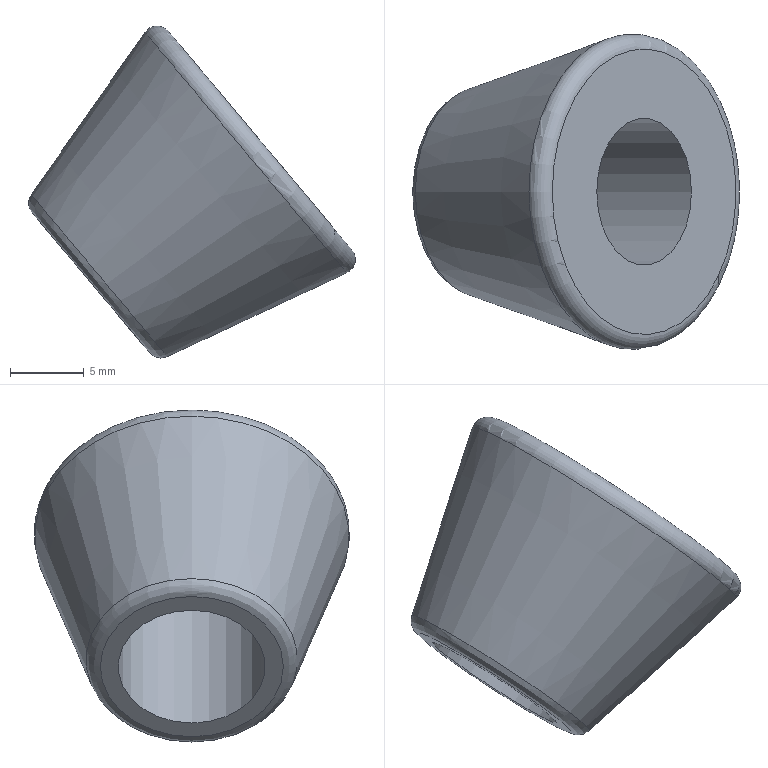Component | NX | HANGERBUSHING | 1 solid | 6 faces | box 22.19 x 21.39 x 22.54 mm | volume 2664 mm3 | plane 2 | torus 2 | cone 1 | cylinder 1 | commonest cylinder face diameters 10 x1
STEP:
#1=CARTESIAN_POINT('',(0.,0.,0.));
#2=DIRECTION('',(0.,0.,1.));
#3=DIRECTION('',(1.,0.,0.));
#4=AXIS2_PLACEMENT_3D('',#1,#2,#3);
#5=CARTESIAN_POINT('',(-451.275,-0.,-55.009));
#6=VERTEX_POINT('',#5);
#7=CARTESIAN_POINT('',(-446.66,-0.,-60.509));
#8=DIRECTION('',(0.766,0.,0.6428));
#9=DIRECTION('',(-0.6428,0.,0.766));
#10=AXIS2_PLACEMENT_3D('',#7,#8,#9);
#11=CIRCLE('',#10,7.179);
#12=CARTESIAN_POINT('',(-435.737,-0.,-51.344));
#13=DIRECTION('',(0.766,0.,0.6428));
#14=DIRECTION('',(-0.6428,0.,0.766));
#15=AXIS2_PLACEMENT_3D('',#12,#13,#14);
#16=CONICAL_SURFACE('',#15,11.,0.2618);
#17=CARTESIAN_POINT('',(0.,-14.259));
#18=DIRECTION('',(1.,0.));
#19=VECTOR('',#18,1.);
#20=LINE('',#17,#19);
#21=(GEOMETRIC_REPRESENTATION_CONTEXT(2)PARAMETRIC_REPRESENTATION_CONTEXT()REPRESENTATION_CONTEXT('',''));
#22=DEFINITIONAL_REPRESENTATION('',(#20),#21);
#23=PCURVE('',#16,#22);
#24=CARTESIAN_POINT('',(-446.462,-0.,-60.343));
#25=DIRECTION('',(0.766,0.,0.6428));
#26=DIRECTION('',(-0.6428,0.,0.766));
#27=AXIS2_PLACEMENT_3D('',#24,#25,#26);
#28=TOROIDAL_SURFACE('',#27,6.213,1.);
#29=CARTESIAN_POINT('',(0.,6.021));
#30=DIRECTION('',(1.,0.));
#31=VECTOR('',#30,1.);
#32=LINE('',#29,#31);
#33=(GEOMETRIC_REPRESENTATION_CONTEXT(2)PARAMETRIC_REPRESENTATION_CONTEXT()REPRESENTATION_CONTEXT('',''));
#34=DEFINITIONAL_REPRESENTATION('',(#32),#33);
#35=PCURVE('',#28,#34);
#36=SURFACE_CURVE('',#11,(#23,#35),.PCURVE_S1.);
#37=EDGE_CURVE('',#6,#6,#36,.T.);
#38=ORIENTED_EDGE('',*,*,#37,.T.);
#39=CARTESIAN_POINT('',(-443.555,-0.,-43.985));
#40=VERTEX_POINT('',#39);
#41=CARTESIAN_POINT('',(-451.275,-0.,-55.009));
#42=CARTESIAN_POINT('',(-443.555,-0.,-43.985));
#43=B_SPLINE_CURVE_WITH_KNOTS('',1,(#41,#42),.UNSPECIFIED.,.F.,.F.,(2,2),(-14.762,-1.303),.PIECEWISE_BEZIER_KNOTS.);
#44=CARTESIAN_POINT('',(6.283,0.));
#45=DIRECTION('',(0.,1.));
#46=VECTOR('',#45,1.);
#47=LINE('',#44,#46);
#48=(GEOMETRIC_REPRESENTATION_CONTEXT(2)PARAMETRIC_REPRESENTATION_CONTEXT()REPRESENTATION_CONTEXT('',''));
#49=DEFINITIONAL_REPRESENTATION('',(#47),#48);
#50=PCURVE('',#16,#49);
#51=CARTESIAN_POINT('',(0.,0.));
#52=DIRECTION('',(0.,1.));
#53=VECTOR('',#52,1.);
#54=LINE('',#51,#53);
#55=(GEOMETRIC_REPRESENTATION_CONTEXT(2)PARAMETRIC_REPRESENTATION_CONTEXT()REPRESENTATION_CONTEXT('',''));
#56=DEFINITIONAL_REPRESENTATION('',(#54),#55);
#57=PCURVE('',#16,#56);
#58=SEAM_CURVE('',#43,(#50,#57),.PCURVE_S1.);
#59=EDGE_CURVE('',#6,#40,#58,.T.);
#60=ORIENTED_EDGE('',*,*,#59,.T.);
#61=CARTESIAN_POINT('',(-429.848,-0.,-60.321));
#62=VERTEX_POINT('',#61);
#63=CARTESIAN_POINT('',(-436.702,-0.,-52.153));
#64=DIRECTION('',(-0.766,0.,-0.6428));
#65=DIRECTION('',(0.6428,0.,-0.766));
#66=AXIS2_PLACEMENT_3D('',#63,#64,#65);
#67=CIRCLE('',#66,10.663);
#68=CARTESIAN_POINT('',(9.425,-1.259));
#69=DIRECTION('',(-1.,0.));
#70=VECTOR('',#69,1.);
#71=LINE('',#68,#70);
#72=(GEOMETRIC_REPRESENTATION_CONTEXT(2)PARAMETRIC_REPRESENTATION_CONTEXT()REPRESENTATION_CONTEXT('',''));
#73=DEFINITIONAL_REPRESENTATION('',(#71),#72);
#74=PCURVE('',#16,#73);
#75=CARTESIAN_POINT('',(-436.503,-0.,-51.987));
#76=DIRECTION('',(0.766,0.,0.6428));
#77=DIRECTION('',(-0.6428,0.,0.766));
#78=AXIS2_PLACEMENT_3D('',#75,#76,#77);
#79=TOROIDAL_SURFACE('',#78,9.697,1.);
#80=CARTESIAN_POINT('',(9.425,6.021));
#81=DIRECTION('',(-1.,-0.));
#82=VECTOR('',#81,1.);
#83=LINE('',#80,#82);
#84=(GEOMETRIC_REPRESENTATION_CONTEXT(2)PARAMETRIC_REPRESENTATION_CONTEXT()REPRESENTATION_CONTEXT('',''));
#85=DEFINITIONAL_REPRESENTATION('',(#83),#84);
#86=PCURVE('',#79,#85);
#87=SURFACE_CURVE('',#67,(#74,#86),.PCURVE_S1.);
#88=EDGE_CURVE('',#40,#62,#87,.T.);
#89=ORIENTED_EDGE('',*,*,#88,.T.);
#90=CARTESIAN_POINT('',(-436.702,-0.,-52.153));
#91=DIRECTION('',(-0.766,0.,-0.6428));
#92=DIRECTION('',(0.6428,0.,-0.766));
#93=AXIS2_PLACEMENT_3D('',#90,#91,#92);
#94=CIRCLE('',#93,10.663);
#95=CARTESIAN_POINT('',(3.142,-1.259));
#96=DIRECTION('',(-1.,0.));
#97=VECTOR('',#96,1.);
#98=LINE('',#95,#97);
#99=(GEOMETRIC_REPRESENTATION_CONTEXT(2)PARAMETRIC_REPRESENTATION_CONTEXT()REPRESENTATION_CONTEXT('',''));
#100=DEFINITIONAL_REPRESENTATION('',(#98),#99);
#101=PCURVE('',#16,#100);
#102=CARTESIAN_POINT('',(3.142,6.021));
#103=DIRECTION('',(-1.,0.));
#104=VECTOR('',#103,1.);
#105=LINE('',#102,#104);
#106=(GEOMETRIC_REPRESENTATION_CONTEXT(2)PARAMETRIC_REPRESENTATION_CONTEXT()REPRESENTATION_CONTEXT('',''));
#107=DEFINITIONAL_REPRESENTATION('',(#105),#106);
#108=PCURVE('',#79,#107);
#109=SURFACE_CURVE('',#94,(#101,#108),.PCURVE_S1.);
#110=EDGE_CURVE('',#62,#40,#109,.T.);
#111=ORIENTED_EDGE('',*,*,#110,.T.);
#112=ORIENTED_EDGE('',*,*,#59,.F.);
#113=EDGE_LOOP('',(#38,#60,#89,#111,#112));
#114=FACE_BOUND('',#113,.T.);
#115=ADVANCED_FACE('',(#114),#16,.T.);
#116=CARTESIAN_POINT('',(-450.442,-0.,-57.155));
#117=VERTEX_POINT('',#116);
#118=CARTESIAN_POINT('',(-447.228,-0.,-60.986));
#119=DIRECTION('',(0.766,0.,0.6428));
#120=DIRECTION('',(-0.6428,0.,0.766));
#121=AXIS2_PLACEMENT_3D('',#118,#119,#120);
#122=CIRCLE('',#121,5.);
#123=CARTESIAN_POINT('',(-447.228,-0.,-60.986));
#124=DIRECTION('',(0.766,0.,0.6428));
#125=DIRECTION('',(-0.6428,0.,0.766));
#126=AXIS2_PLACEMENT_3D('',#123,#124,#125);
#127=PLANE('',#126);
#128=CARTESIAN_POINT('',(0.,0.));
#129=DIRECTION('',(1.,0.));
#130=AXIS2_PLACEMENT_2D('',#128,#129);
#131=CIRCLE('',#130,5.);
#132=(GEOMETRIC_REPRESENTATION_CONTEXT(2)PARAMETRIC_REPRESENTATION_CONTEXT()REPRESENTATION_CONTEXT('',''));
#133=DEFINITIONAL_REPRESENTATION('',(#131),#132);
#134=PCURVE('',#127,#133);
#135=CARTESIAN_POINT('',(-447.228,-0.,-60.986));
#136=DIRECTION('',(0.766,0.,0.6428));
#137=DIRECTION('',(-0.6428,0.,0.766));
#138=AXIS2_PLACEMENT_3D('',#135,#136,#137);
#139=CYLINDRICAL_SURFACE('',#138,5.);
#140=CARTESIAN_POINT('',(0.,0.));
#141=DIRECTION('',(1.,0.));
#142=VECTOR('',#141,1.);
#143=LINE('',#140,#142);
#144=(GEOMETRIC_REPRESENTATION_CONTEXT(2)PARAMETRIC_REPRESENTATION_CONTEXT()REPRESENTATION_CONTEXT('',''));
#145=DEFINITIONAL_REPRESENTATION('',(#143),#144);
#146=PCURVE('',#139,#145);
#147=SURFACE_CURVE('',#122,(#134,#146),.PCURVE_S1.);
#148=EDGE_CURVE('',#117,#117,#147,.T.);
#149=ORIENTED_EDGE('',*,*,#148,.T.);
#150=EDGE_LOOP('',(#149));
#151=FACE_BOUND('',#150,.T.);
#152=CARTESIAN_POINT('',(-451.222,-0.,-56.226));
#153=VERTEX_POINT('',#152);
#154=CARTESIAN_POINT('',(-447.228,-0.,-60.986));
#155=DIRECTION('',(-0.766,0.,-0.6428));
#156=DIRECTION('',(-0.6428,0.,0.766));
#157=AXIS2_PLACEMENT_3D('',#154,#155,#156);
#158=CIRCLE('',#157,6.213);
#159=CARTESIAN_POINT('',(6.213,0.));
#160=CARTESIAN_POINT('',(6.213,-10.762));
#161=CARTESIAN_POINT('',(-3.107,-5.381));
#162=CARTESIAN_POINT('',(-12.427,-0.));
#163=CARTESIAN_POINT('',(-3.107,5.381));
#164=CARTESIAN_POINT('',(6.213,10.762));
#165=CARTESIAN_POINT('',(6.213,0.));
#166=(BOUNDED_CURVE()B_SPLINE_CURVE(2,(#159,#160,#161,#162,#163,#164,#165),.UNSPECIFIED.,.T.,.F.)B_SPLINE_CURVE_WITH_KNOTS((1,2,2,2,2,1),(-2.094,0.,2.094,4.189,6.283,8.378),.UNSPECIFIED.)CURVE()GEOMETRIC_REPRESENTATION_ITEM()RATIONAL_B_SPLINE_CURVE((1.,0.5,1.,0.5,1.,0.5,1.))REPRESENTATION_ITEM(''));
#167=(GEOMETRIC_REPRESENTATION_CONTEXT(2)PARAMETRIC_REPRESENTATION_CONTEXT()REPRESENTATION_CONTEXT('',''));
#168=DEFINITIONAL_REPRESENTATION('',(#166),#167);
#169=PCURVE('',#127,#168);
#170=CARTESIAN_POINT('',(6.283,4.712));
#171=DIRECTION('',(-1.,0.));
#172=VECTOR('',#171,1.);
#173=LINE('',#170,#172);
#174=(GEOMETRIC_REPRESENTATION_CONTEXT(2)PARAMETRIC_REPRESENTATION_CONTEXT()REPRESENTATION_CONTEXT('',''));
#175=DEFINITIONAL_REPRESENTATION('',(#173),#174);
#176=PCURVE('',#28,#175);
#177=SURFACE_CURVE('',#158,(#169,#176),.PCURVE_S1.);
#178=EDGE_CURVE('',#153,#153,#177,.T.);
#179=ORIENTED_EDGE('',*,*,#178,.T.);
#180=EDGE_LOOP('',(#179));
#181=FACE_BOUND('',#180,.T.);
#182=ADVANCED_FACE('',(#151,#181),#127,.F.);
#183=CARTESIAN_POINT('',(-438.951,-0.,-47.514));
#184=VERTEX_POINT('',#183);
#185=CARTESIAN_POINT('',(-435.737,-0.,-51.344));
#186=DIRECTION('',(0.766,0.,0.6428));
#187=DIRECTION('',(-0.6428,0.,0.766));
#188=AXIS2_PLACEMENT_3D('',#185,#186,#187);
#189=CIRCLE('',#188,5.);
#190=CARTESIAN_POINT('',(-435.737,-0.,-51.344));
#191=DIRECTION('',(0.766,0.,0.6428));
#192=DIRECTION('',(-0.6428,0.,0.766));
#193=AXIS2_PLACEMENT_3D('',#190,#191,#192);
#194=PLANE('',#193);
#195=CARTESIAN_POINT('',(0.,0.));
#196=DIRECTION('',(1.,0.));
#197=AXIS2_PLACEMENT_2D('',#195,#196);
#198=CIRCLE('',#197,5.);
#199=(GEOMETRIC_REPRESENTATION_CONTEXT(2)PARAMETRIC_REPRESENTATION_CONTEXT()REPRESENTATION_CONTEXT('',''));
#200=DEFINITIONAL_REPRESENTATION('',(#198),#199);
#201=PCURVE('',#194,#200);
#202=CARTESIAN_POINT('',(0.,15.));
#203=DIRECTION('',(1.,0.));
#204=VECTOR('',#203,1.);
#205=LINE('',#202,#204);
#206=(GEOMETRIC_REPRESENTATION_CONTEXT(2)PARAMETRIC_REPRESENTATION_CONTEXT()REPRESENTATION_CONTEXT('',''));
#207=DEFINITIONAL_REPRESENTATION('',(#205),#206);
#208=PCURVE('',#139,#207);
#209=SURFACE_CURVE('',#189,(#201,#208),.PCURVE_S1.);
#210=EDGE_CURVE('',#184,#184,#209,.T.);
#211=ORIENTED_EDGE('',*,*,#210,.F.);
#212=EDGE_LOOP('',(#211));
#213=FACE_BOUND('',#212,.T.);
#214=CARTESIAN_POINT('',(-441.97,-0.,-43.916));
#215=VERTEX_POINT('',#214);
#216=CARTESIAN_POINT('',(-435.737,-0.,-51.344));
#217=DIRECTION('',(0.766,0.,0.6428));
#218=DIRECTION('',(-0.6428,0.,0.766));
#219=AXIS2_PLACEMENT_3D('',#216,#217,#218);
#220=CIRCLE('',#219,9.697);
#221=CARTESIAN_POINT('',(0.,0.));
#222=DIRECTION('',(1.,0.));
#223=AXIS2_PLACEMENT_2D('',#221,#222);
#224=CIRCLE('',#223,9.697);
#225=(GEOMETRIC_REPRESENTATION_CONTEXT(2)PARAMETRIC_REPRESENTATION_CONTEXT()REPRESENTATION_CONTEXT('',''));
#226=DEFINITIONAL_REPRESENTATION('',(#224),#225);
#227=PCURVE('',#194,#226);
#228=CARTESIAN_POINT('',(0.,7.854));
#229=DIRECTION('',(1.,0.));
#230=VECTOR('',#229,1.);
#231=LINE('',#228,#230);
#232=(GEOMETRIC_REPRESENTATION_CONTEXT(2)PARAMETRIC_REPRESENTATION_CONTEXT()REPRESENTATION_CONTEXT('',''));
#233=DEFINITIONAL_REPRESENTATION('',(#231),#232);
#234=PCURVE('',#79,#233);
#235=SURFACE_CURVE('',#220,(#227,#234),.PCURVE_S1.);
#236=EDGE_CURVE('',#215,#215,#235,.T.);
#237=ORIENTED_EDGE('',*,*,#236,.T.);
#238=EDGE_LOOP('',(#237));
#239=FACE_BOUND('',#238,.T.);
#240=ADVANCED_FACE('',(#213,#239),#194,.T.);
#241=ORIENTED_EDGE('',*,*,#37,.F.);
#242=CARTESIAN_POINT('',(-451.222,-0.,-56.226));
#243=CARTESIAN_POINT('',(-451.364,-0.,-56.056));
#244=CARTESIAN_POINT('',(-451.459,-0.,-55.852));
#245=CARTESIAN_POINT('',(-451.498,-0.,-55.629));
#246=CARTESIAN_POINT('',(-451.479,-0.,-55.402));
#247=CARTESIAN_POINT('',(-451.402,-0.,-55.191));
#248=CARTESIAN_POINT('',(-451.275,-0.,-55.009));
#249=(BOUNDED_CURVE()B_SPLINE_CURVE(6,(#242,#243,#244,#245,#246,#247,#248),.UNSPECIFIED.,.F.,.F.)B_SPLINE_CURVE_WITH_KNOTS((7,7),(4.712,6.021),.PIECEWISE_BEZIER_KNOTS.)CURVE()GEOMETRIC_REPRESENTATION_ITEM()RATIONAL_B_SPLINE_CURVE((1.022,1.007,0.9986,0.9958,0.9986,1.007,1.022))REPRESENTATION_ITEM(''));
#250=CARTESIAN_POINT('',(0.,0.));
#251=DIRECTION('',(0.,1.));
#252=VECTOR('',#251,1.);
#253=LINE('',#250,#252);
#254=(GEOMETRIC_REPRESENTATION_CONTEXT(2)PARAMETRIC_REPRESENTATION_CONTEXT()REPRESENTATION_CONTEXT('',''));
#255=DEFINITIONAL_REPRESENTATION('',(#253),#254);
#256=PCURVE('',#28,#255);
#257=CARTESIAN_POINT('',(6.283,0.));
#258=DIRECTION('',(0.,1.));
#259=VECTOR('',#258,1.);
#260=LINE('',#257,#259);
#261=(GEOMETRIC_REPRESENTATION_CONTEXT(2)PARAMETRIC_REPRESENTATION_CONTEXT()REPRESENTATION_CONTEXT('',''));
#262=DEFINITIONAL_REPRESENTATION('',(#260),#261);
#263=PCURVE('',#28,#262);
#264=SEAM_CURVE('',#249,(#256,#263),.PCURVE_S1.);
#265=EDGE_CURVE('',#153,#6,#264,.T.);
#266=ORIENTED_EDGE('',*,*,#265,.F.);
#267=ORIENTED_EDGE('',*,*,#178,.F.);
#268=ORIENTED_EDGE('',*,*,#265,.T.);
#269=EDGE_LOOP('',(#241,#266,#267,#268));
#270=FACE_BOUND('',#269,.T.);
#271=ADVANCED_FACE('',(#270),#28,.T.);
#272=ORIENTED_EDGE('',*,*,#110,.F.);
#273=ORIENTED_EDGE('',*,*,#88,.F.);
#274=CARTESIAN_POINT('',(-443.555,-0.,-43.985));
#275=CARTESIAN_POINT('',(-443.38,-0.,-43.735));
#276=CARTESIAN_POINT('',(-443.113,-0.,-43.549));
#277=CARTESIAN_POINT('',(-442.784,-0.,-43.469));
#278=CARTESIAN_POINT('',(-442.449,-0.,-43.52));
#279=CARTESIAN_POINT('',(-442.167,-0.,-43.682));
#280=CARTESIAN_POINT('',(-441.97,-0.,-43.916));
#281=B_SPLINE_CURVE_WITH_KNOTS('',6,(#274,#275,#276,#277,#278,#279,#280),.UNSPECIFIED.,.F.,.F.,(7,7),(6.021,7.854),.PIECEWISE_BEZIER_KNOTS.);
#282=CARTESIAN_POINT('',(6.283,0.));
#283=DIRECTION('',(0.,1.));
#284=VECTOR('',#283,1.);
#285=LINE('',#282,#284);
#286=(GEOMETRIC_REPRESENTATION_CONTEXT(2)PARAMETRIC_REPRESENTATION_CONTEXT()REPRESENTATION_CONTEXT('',''));
#287=DEFINITIONAL_REPRESENTATION('',(#285),#286);
#288=PCURVE('',#79,#287);
#289=CARTESIAN_POINT('',(0.,0.));
#290=DIRECTION('',(0.,1.));
#291=VECTOR('',#290,1.);
#292=LINE('',#289,#291);
#293=(GEOMETRIC_REPRESENTATION_CONTEXT(2)PARAMETRIC_REPRESENTATION_CONTEXT()REPRESENTATION_CONTEXT('',''));
#294=DEFINITIONAL_REPRESENTATION('',(#292),#293);
#295=PCURVE('',#79,#294);
#296=SEAM_CURVE('',#281,(#288,#295),.PCURVE_S1.);
#297=EDGE_CURVE('',#40,#215,#296,.T.);
#298=ORIENTED_EDGE('',*,*,#297,.T.);
#299=ORIENTED_EDGE('',*,*,#236,.F.);
#300=ORIENTED_EDGE('',*,*,#297,.F.);
#301=EDGE_LOOP('',(#272,#273,#298,#299,#300));
#302=FACE_BOUND('',#301,.T.);
#303=ADVANCED_FACE('',(#302),#79,.T.);
#304=ORIENTED_EDGE('',*,*,#210,.F.);
#305=CARTESIAN_POINT('',(-450.442,-0.,-57.155));
#306=CARTESIAN_POINT('',(-438.951,-0.,-47.514));
#307=B_SPLINE_CURVE_WITH_KNOTS('',1,(#305,#306),.UNSPECIFIED.,.F.,.F.,(2,2),(0.,15.),.PIECEWISE_BEZIER_KNOTS.);
#308=CARTESIAN_POINT('',(0.,0.));
#309=DIRECTION('',(0.,1.));
#310=VECTOR('',#309,1.);
#311=LINE('',#308,#310);
#312=(GEOMETRIC_REPRESENTATION_CONTEXT(2)PARAMETRIC_REPRESENTATION_CONTEXT()REPRESENTATION_CONTEXT('',''));
#313=DEFINITIONAL_REPRESENTATION('',(#311),#312);
#314=PCURVE('',#139,#313);
#315=CARTESIAN_POINT('',(6.283,0.));
#316=DIRECTION('',(0.,1.));
#317=VECTOR('',#316,1.);
#318=LINE('',#315,#317);
#319=(GEOMETRIC_REPRESENTATION_CONTEXT(2)PARAMETRIC_REPRESENTATION_CONTEXT()REPRESENTATION_CONTEXT('',''));
#320=DEFINITIONAL_REPRESENTATION('',(#318),#319);
#321=PCURVE('',#139,#320);
#322=SEAM_CURVE('',#307,(#314,#321),.PCURVE_S1.);
#323=EDGE_CURVE('',#117,#184,#322,.T.);
#324=ORIENTED_EDGE('',*,*,#323,.F.);
#325=ORIENTED_EDGE('',*,*,#148,.T.);
#326=ORIENTED_EDGE('',*,*,#323,.T.);
#327=EDGE_LOOP('',(#304,#324,#325,#326));
#328=FACE_BOUND('',#327,.F.);
#329=ADVANCED_FACE('',(#328),#139,.F.);
#330=CLOSED_SHELL('',(#115,#182,#240,#271,#303,#329));
#331=MANIFOLD_SOLID_BREP('',#330);
#332=(LENGTH_UNIT()NAMED_UNIT(*)SI_UNIT(.MILLI.,.METRE.));
#333=UNCERTAINTY_MEASURE_WITH_UNIT(LENGTH_MEASURE(0.00001),#332,'','');
#334=(NAMED_UNIT(*)PLANE_ANGLE_UNIT()SI_UNIT($,.RADIAN.));
#335=(NAMED_UNIT(*)SI_UNIT($,.STERADIAN.)SOLID_ANGLE_UNIT());
#336=(GEOMETRIC_REPRESENTATION_CONTEXT(3)GLOBAL_UNCERTAINTY_ASSIGNED_CONTEXT((#333))GLOBAL_UNIT_ASSIGNED_CONTEXT((#332,#334,#335))REPRESENTATION_CONTEXT('',''));
#337=ADVANCED_BREP_SHAPE_REPRESENTATION('',(#4,#331),#336);